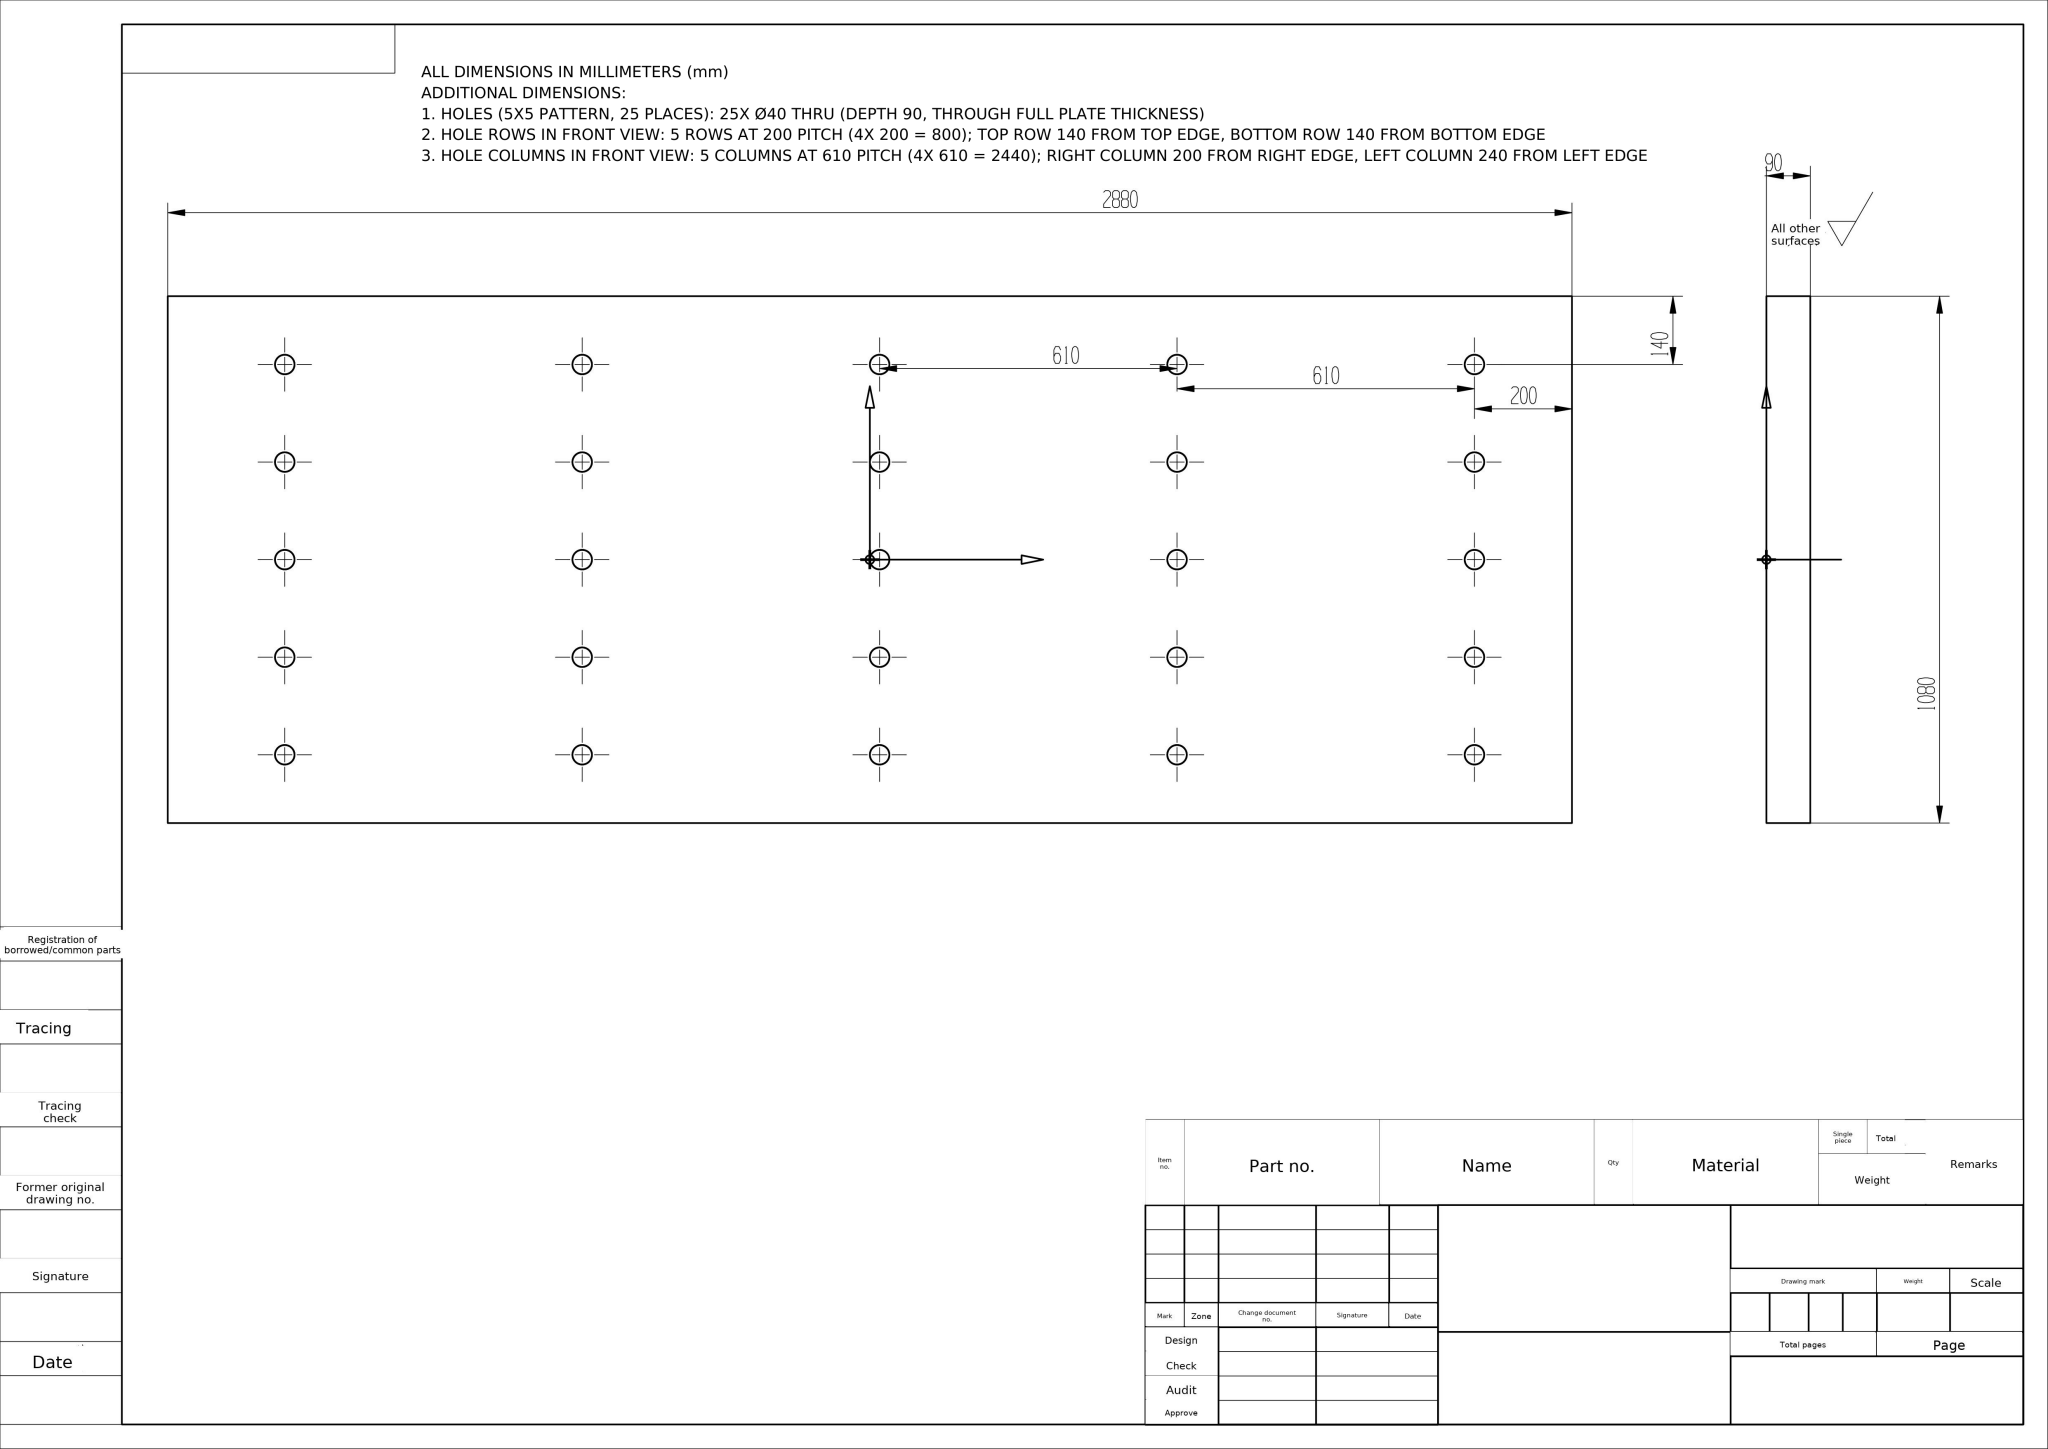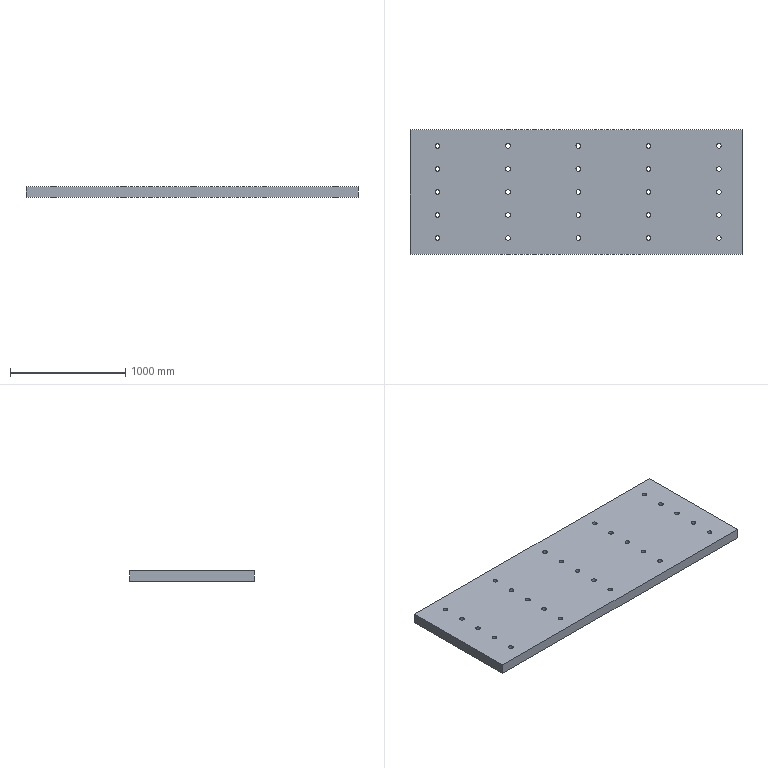Part | NX | mm | 1 solid | 31 faces | box 2880 x 1080 x 90 mm | volume 277108567 mm3 | cylinder 25 | plane 6 | commonest cylinder face diameters 40 x25
STEP:
#1=CARTESIAN_POINT('',(0.,0.,0.));
#2=DIRECTION('',(0.,0.,1.));
#3=DIRECTION('',(1.,0.,0.));
#4=AXIS2_PLACEMENT_3D('',#1,#2,#3);
#5=(LENGTH_UNIT()NAMED_UNIT(*)SI_UNIT(.MILLI.,.METRE.));
#6=UNCERTAINTY_MEASURE_WITH_UNIT(LENGTH_MEASURE(0.00002),#5,'','');
#7=(NAMED_UNIT(*)PLANE_ANGLE_UNIT()SI_UNIT($,.RADIAN.));
#8=PLANE_ANGLE_MEASURE_WITH_UNIT(PLANE_ANGLE_MEASURE(0.01745),#7);
#9=DIMENSIONAL_EXPONENTS(0.,0.,0.,0.,0.,0.,0.);
#10=(CONVERSION_BASED_UNIT('',#8)NAMED_UNIT(#9)PLANE_ANGLE_UNIT());
#11=(NAMED_UNIT(*)SI_UNIT($,.STERADIAN.)SOLID_ANGLE_UNIT());
#12=(GEOMETRIC_REPRESENTATION_CONTEXT(3)GLOBAL_UNCERTAINTY_ASSIGNED_CONTEXT((#6))GLOBAL_UNIT_ASSIGNED_CONTEXT((#5,#10,#11))REPRESENTATION_CONTEXT('',''));
#13=SHAPE_REPRESENTATION('',(#4),#12);
#14=CARTESIAN_POINT('',(-1440.,540.,0.));
#15=VERTEX_POINT('',#14);
#16=CARTESIAN_POINT('',(-1440.,-540.,0.));
#17=VERTEX_POINT('',#16);
#18=CARTESIAN_POINT('',(-1440.,540.,0.));
#19=DIRECTION('',(-0.,-1.,0.));
#20=VECTOR('',#19,1.);
#21=LINE('',#18,#20);
#22=EDGE_CURVE('',#15,#17,#21,.T.);
#23=ORIENTED_EDGE('',*,*,#22,.T.);
#24=CARTESIAN_POINT('',(-1440.,-540.,90.));
#25=VERTEX_POINT('',#24);
#26=CARTESIAN_POINT('',(-1440.,-540.,90.));
#27=DIRECTION('',(0.,0.,-1.));
#28=VECTOR('',#27,1.);
#29=LINE('',#26,#28);
#30=EDGE_CURVE('',#25,#17,#29,.T.);
#31=ORIENTED_EDGE('',*,*,#30,.F.);
#32=CARTESIAN_POINT('',(-1440.,540.,90.));
#33=VERTEX_POINT('',#32);
#34=CARTESIAN_POINT('',(-1440.,540.,90.));
#35=DIRECTION('',(-0.,-1.,0.));
#36=VECTOR('',#35,1.);
#37=LINE('',#34,#36);
#38=EDGE_CURVE('',#33,#25,#37,.T.);
#39=ORIENTED_EDGE('',*,*,#38,.F.);
#40=CARTESIAN_POINT('',(-1440.,540.,90.));
#41=DIRECTION('',(0.,0.,-1.));
#42=VECTOR('',#41,1.);
#43=LINE('',#40,#42);
#44=EDGE_CURVE('',#33,#15,#43,.T.);
#45=ORIENTED_EDGE('',*,*,#44,.T.);
#46=EDGE_LOOP('',(#23,#31,#39,#45));
#47=FACE_OUTER_BOUND('',#46,.T.);
#48=CARTESIAN_POINT('',(-1440.,540.,90.));
#49=DIRECTION('',(1.,-0.,0.));
#50=DIRECTION('',(0.,1.,0.));
#51=AXIS2_PLACEMENT_3D('',#48,#49,#50);
#52=PLANE('',#51);
#53=ADVANCED_FACE('',(#47),#52,.F.);
#54=CARTESIAN_POINT('',(1440.,-540.,0.));
#55=VERTEX_POINT('',#54);
#56=CARTESIAN_POINT('',(-1440.,-540.,0.));
#57=DIRECTION('',(1.,0.,0.));
#58=VECTOR('',#57,1.);
#59=LINE('',#56,#58);
#60=EDGE_CURVE('',#17,#55,#59,.T.);
#61=ORIENTED_EDGE('',*,*,#60,.T.);
#62=CARTESIAN_POINT('',(1440.,-540.,90.));
#63=VERTEX_POINT('',#62);
#64=CARTESIAN_POINT('',(1440.,-540.,90.));
#65=DIRECTION('',(0.,0.,-1.));
#66=VECTOR('',#65,1.);
#67=LINE('',#64,#66);
#68=EDGE_CURVE('',#63,#55,#67,.T.);
#69=ORIENTED_EDGE('',*,*,#68,.F.);
#70=CARTESIAN_POINT('',(-1440.,-540.,90.));
#71=DIRECTION('',(1.,0.,0.));
#72=VECTOR('',#71,1.);
#73=LINE('',#70,#72);
#74=EDGE_CURVE('',#25,#63,#73,.T.);
#75=ORIENTED_EDGE('',*,*,#74,.F.);
#76=ORIENTED_EDGE('',*,*,#30,.T.);
#77=EDGE_LOOP('',(#61,#69,#75,#76));
#78=FACE_OUTER_BOUND('',#77,.T.);
#79=CARTESIAN_POINT('',(-1440.,-540.,90.));
#80=DIRECTION('',(0.,1.,0.));
#81=DIRECTION('',(0.,0.,1.));
#82=AXIS2_PLACEMENT_3D('',#79,#80,#81);
#83=PLANE('',#82);
#84=ADVANCED_FACE('',(#78),#83,.F.);
#85=CARTESIAN_POINT('',(1440.,540.,0.));
#86=VERTEX_POINT('',#85);
#87=CARTESIAN_POINT('',(1440.,-540.,0.));
#88=DIRECTION('',(0.,1.,0.));
#89=VECTOR('',#88,1.);
#90=LINE('',#87,#89);
#91=EDGE_CURVE('',#55,#86,#90,.T.);
#92=ORIENTED_EDGE('',*,*,#91,.T.);
#93=CARTESIAN_POINT('',(1440.,540.,90.));
#94=VERTEX_POINT('',#93);
#95=CARTESIAN_POINT('',(1440.,540.,90.));
#96=DIRECTION('',(0.,0.,-1.));
#97=VECTOR('',#96,1.);
#98=LINE('',#95,#97);
#99=EDGE_CURVE('',#94,#86,#98,.T.);
#100=ORIENTED_EDGE('',*,*,#99,.F.);
#101=CARTESIAN_POINT('',(1440.,-540.,90.));
#102=DIRECTION('',(0.,1.,0.));
#103=VECTOR('',#102,1.);
#104=LINE('',#101,#103);
#105=EDGE_CURVE('',#63,#94,#104,.T.);
#106=ORIENTED_EDGE('',*,*,#105,.F.);
#107=ORIENTED_EDGE('',*,*,#68,.T.);
#108=EDGE_LOOP('',(#92,#100,#106,#107));
#109=FACE_OUTER_BOUND('',#108,.T.);
#110=CARTESIAN_POINT('',(1440.,-540.,90.));
#111=DIRECTION('',(-1.,0.,0.));
#112=DIRECTION('',(0.,0.,1.));
#113=AXIS2_PLACEMENT_3D('',#110,#111,#112);
#114=PLANE('',#113);
#115=ADVANCED_FACE('',(#109),#114,.F.);
#116=CARTESIAN_POINT('',(1260.,200.,90.));
#117=VERTEX_POINT('',#116);
#118=CARTESIAN_POINT('',(1240.,200.,90.));
#119=DIRECTION('',(0.,0.,1.));
#120=DIRECTION('',(1.,0.,0.));
#121=AXIS2_PLACEMENT_3D('',#118,#119,#120);
#122=CIRCLE('',#121,20.);
#123=EDGE_CURVE('',#117,#117,#122,.T.);
#124=ORIENTED_EDGE('',*,*,#123,.T.);
#125=EDGE_LOOP('',(#124));
#126=FACE_BOUND('',#125,.T.);
#127=CARTESIAN_POINT('',(1260.,200.,0.));
#128=VERTEX_POINT('',#127);
#129=CARTESIAN_POINT('',(1240.,200.,0.));
#130=DIRECTION('',(0.,0.,1.));
#131=DIRECTION('',(1.,0.,0.));
#132=AXIS2_PLACEMENT_3D('',#129,#130,#131);
#133=CIRCLE('',#132,20.);
#134=EDGE_CURVE('',#128,#128,#133,.T.);
#135=ORIENTED_EDGE('',*,*,#134,.F.);
#136=EDGE_LOOP('',(#135));
#137=FACE_BOUND('',#136,.T.);
#138=CARTESIAN_POINT('',(1240.,200.,90.));
#139=DIRECTION('',(0.,0.,-1.));
#140=DIRECTION('',(-1.,0.,0.));
#141=AXIS2_PLACEMENT_3D('',#138,#139,#140);
#142=CYLINDRICAL_SURFACE('',#141,20.);
#143=ADVANCED_FACE('',(#126,#137),#142,.F.);
#144=CARTESIAN_POINT('',(1260.,-0.,90.));
#145=VERTEX_POINT('',#144);
#146=CARTESIAN_POINT('',(1240.,-0.,90.));
#147=DIRECTION('',(0.,0.,1.));
#148=DIRECTION('',(1.,0.,0.));
#149=AXIS2_PLACEMENT_3D('',#146,#147,#148);
#150=CIRCLE('',#149,20.);
#151=EDGE_CURVE('',#145,#145,#150,.T.);
#152=ORIENTED_EDGE('',*,*,#151,.T.);
#153=EDGE_LOOP('',(#152));
#154=FACE_BOUND('',#153,.T.);
#155=CARTESIAN_POINT('',(1260.,-0.,0.));
#156=VERTEX_POINT('',#155);
#157=CARTESIAN_POINT('',(1240.,-0.,0.));
#158=DIRECTION('',(0.,0.,1.));
#159=DIRECTION('',(1.,0.,0.));
#160=AXIS2_PLACEMENT_3D('',#157,#158,#159);
#161=CIRCLE('',#160,20.);
#162=EDGE_CURVE('',#156,#156,#161,.T.);
#163=ORIENTED_EDGE('',*,*,#162,.F.);
#164=EDGE_LOOP('',(#163));
#165=FACE_BOUND('',#164,.T.);
#166=CARTESIAN_POINT('',(1240.,-0.,90.));
#167=DIRECTION('',(0.,0.,-1.));
#168=DIRECTION('',(-1.,0.,0.));
#169=AXIS2_PLACEMENT_3D('',#166,#167,#168);
#170=CYLINDRICAL_SURFACE('',#169,20.);
#171=ADVANCED_FACE('',(#154,#165),#170,.F.);
#172=CARTESIAN_POINT('',(1260.,-200.,90.));
#173=VERTEX_POINT('',#172);
#174=CARTESIAN_POINT('',(1240.,-200.,90.));
#175=DIRECTION('',(0.,0.,1.));
#176=DIRECTION('',(1.,0.,0.));
#177=AXIS2_PLACEMENT_3D('',#174,#175,#176);
#178=CIRCLE('',#177,20.);
#179=EDGE_CURVE('',#173,#173,#178,.T.);
#180=ORIENTED_EDGE('',*,*,#179,.T.);
#181=EDGE_LOOP('',(#180));
#182=FACE_BOUND('',#181,.T.);
#183=CARTESIAN_POINT('',(1260.,-200.,0.));
#184=VERTEX_POINT('',#183);
#185=CARTESIAN_POINT('',(1240.,-200.,0.));
#186=DIRECTION('',(0.,0.,1.));
#187=DIRECTION('',(1.,0.,0.));
#188=AXIS2_PLACEMENT_3D('',#185,#186,#187);
#189=CIRCLE('',#188,20.);
#190=EDGE_CURVE('',#184,#184,#189,.T.);
#191=ORIENTED_EDGE('',*,*,#190,.F.);
#192=EDGE_LOOP('',(#191));
#193=FACE_BOUND('',#192,.T.);
#194=CARTESIAN_POINT('',(1240.,-200.,90.));
#195=DIRECTION('',(0.,0.,-1.));
#196=DIRECTION('',(-1.,0.,0.));
#197=AXIS2_PLACEMENT_3D('',#194,#195,#196);
#198=CYLINDRICAL_SURFACE('',#197,20.);
#199=ADVANCED_FACE('',(#182,#193),#198,.F.);
#200=CARTESIAN_POINT('',(1260.,-400.,90.));
#201=VERTEX_POINT('',#200);
#202=CARTESIAN_POINT('',(1240.,-400.,90.));
#203=DIRECTION('',(0.,0.,1.));
#204=DIRECTION('',(1.,0.,0.));
#205=AXIS2_PLACEMENT_3D('',#202,#203,#204);
#206=CIRCLE('',#205,20.);
#207=EDGE_CURVE('',#201,#201,#206,.T.);
#208=ORIENTED_EDGE('',*,*,#207,.T.);
#209=EDGE_LOOP('',(#208));
#210=FACE_BOUND('',#209,.T.);
#211=CARTESIAN_POINT('',(1260.,-400.,0.));
#212=VERTEX_POINT('',#211);
#213=CARTESIAN_POINT('',(1240.,-400.,0.));
#214=DIRECTION('',(0.,0.,1.));
#215=DIRECTION('',(1.,0.,0.));
#216=AXIS2_PLACEMENT_3D('',#213,#214,#215);
#217=CIRCLE('',#216,20.);
#218=EDGE_CURVE('',#212,#212,#217,.T.);
#219=ORIENTED_EDGE('',*,*,#218,.F.);
#220=EDGE_LOOP('',(#219));
#221=FACE_BOUND('',#220,.T.);
#222=CARTESIAN_POINT('',(1240.,-400.,90.));
#223=DIRECTION('',(0.,0.,-1.));
#224=DIRECTION('',(-1.,0.,0.));
#225=AXIS2_PLACEMENT_3D('',#222,#223,#224);
#226=CYLINDRICAL_SURFACE('',#225,20.);
#227=ADVANCED_FACE('',(#210,#221),#226,.F.);
#228=CARTESIAN_POINT('',(650.,400.,90.));
#229=VERTEX_POINT('',#228);
#230=CARTESIAN_POINT('',(630.,400.,90.));
#231=DIRECTION('',(0.,0.,1.));
#232=DIRECTION('',(1.,0.,0.));
#233=AXIS2_PLACEMENT_3D('',#230,#231,#232);
#234=CIRCLE('',#233,20.);
#235=EDGE_CURVE('',#229,#229,#234,.T.);
#236=ORIENTED_EDGE('',*,*,#235,.T.);
#237=EDGE_LOOP('',(#236));
#238=FACE_BOUND('',#237,.T.);
#239=CARTESIAN_POINT('',(650.,400.,0.));
#240=VERTEX_POINT('',#239);
#241=CARTESIAN_POINT('',(630.,400.,0.));
#242=DIRECTION('',(0.,0.,1.));
#243=DIRECTION('',(1.,0.,0.));
#244=AXIS2_PLACEMENT_3D('',#241,#242,#243);
#245=CIRCLE('',#244,20.);
#246=EDGE_CURVE('',#240,#240,#245,.T.);
#247=ORIENTED_EDGE('',*,*,#246,.F.);
#248=EDGE_LOOP('',(#247));
#249=FACE_BOUND('',#248,.T.);
#250=CARTESIAN_POINT('',(630.,400.,90.));
#251=DIRECTION('',(0.,0.,-1.));
#252=DIRECTION('',(-1.,0.,0.));
#253=AXIS2_PLACEMENT_3D('',#250,#251,#252);
#254=CYLINDRICAL_SURFACE('',#253,20.);
#255=ADVANCED_FACE('',(#238,#249),#254,.F.);
#256=CARTESIAN_POINT('',(650.,200.,90.));
#257=VERTEX_POINT('',#256);
#258=CARTESIAN_POINT('',(630.,200.,90.));
#259=DIRECTION('',(0.,0.,1.));
#260=DIRECTION('',(1.,0.,0.));
#261=AXIS2_PLACEMENT_3D('',#258,#259,#260);
#262=CIRCLE('',#261,20.);
#263=EDGE_CURVE('',#257,#257,#262,.T.);
#264=ORIENTED_EDGE('',*,*,#263,.T.);
#265=EDGE_LOOP('',(#264));
#266=FACE_BOUND('',#265,.T.);
#267=CARTESIAN_POINT('',(650.,200.,0.));
#268=VERTEX_POINT('',#267);
#269=CARTESIAN_POINT('',(630.,200.,0.));
#270=DIRECTION('',(0.,0.,1.));
#271=DIRECTION('',(1.,0.,0.));
#272=AXIS2_PLACEMENT_3D('',#269,#270,#271);
#273=CIRCLE('',#272,20.);
#274=EDGE_CURVE('',#268,#268,#273,.T.);
#275=ORIENTED_EDGE('',*,*,#274,.F.);
#276=EDGE_LOOP('',(#275));
#277=FACE_BOUND('',#276,.T.);
#278=CARTESIAN_POINT('',(630.,200.,90.));
#279=DIRECTION('',(0.,0.,-1.));
#280=DIRECTION('',(-1.,0.,0.));
#281=AXIS2_PLACEMENT_3D('',#278,#279,#280);
#282=CYLINDRICAL_SURFACE('',#281,20.);
#283=ADVANCED_FACE('',(#266,#277),#282,.F.);
#284=CARTESIAN_POINT('',(650.,-0.,90.));
#285=VERTEX_POINT('',#284);
#286=CARTESIAN_POINT('',(630.,-0.,90.));
#287=DIRECTION('',(0.,0.,1.));
#288=DIRECTION('',(1.,0.,0.));
#289=AXIS2_PLACEMENT_3D('',#286,#287,#288);
#290=CIRCLE('',#289,20.);
#291=EDGE_CURVE('',#285,#285,#290,.T.);
#292=ORIENTED_EDGE('',*,*,#291,.T.);
#293=EDGE_LOOP('',(#292));
#294=FACE_BOUND('',#293,.T.);
#295=CARTESIAN_POINT('',(650.,-0.,0.));
#296=VERTEX_POINT('',#295);
#297=CARTESIAN_POINT('',(630.,-0.,0.));
#298=DIRECTION('',(0.,0.,1.));
#299=DIRECTION('',(1.,0.,0.));
#300=AXIS2_PLACEMENT_3D('',#297,#298,#299);
#301=CIRCLE('',#300,20.);
#302=EDGE_CURVE('',#296,#296,#301,.T.);
#303=ORIENTED_EDGE('',*,*,#302,.F.);
#304=EDGE_LOOP('',(#303));
#305=FACE_BOUND('',#304,.T.);
#306=CARTESIAN_POINT('',(630.,-0.,90.));
#307=DIRECTION('',(0.,0.,-1.));
#308=DIRECTION('',(-1.,0.,0.));
#309=AXIS2_PLACEMENT_3D('',#306,#307,#308);
#310=CYLINDRICAL_SURFACE('',#309,20.);
#311=ADVANCED_FACE('',(#294,#305),#310,.F.);
#312=CARTESIAN_POINT('',(650.,-200.,90.));
#313=VERTEX_POINT('',#312);
#314=CARTESIAN_POINT('',(630.,-200.,90.));
#315=DIRECTION('',(0.,0.,1.));
#316=DIRECTION('',(1.,0.,0.));
#317=AXIS2_PLACEMENT_3D('',#314,#315,#316);
#318=CIRCLE('',#317,20.);
#319=EDGE_CURVE('',#313,#313,#318,.T.);
#320=ORIENTED_EDGE('',*,*,#319,.T.);
#321=EDGE_LOOP('',(#320));
#322=FACE_BOUND('',#321,.T.);
#323=CARTESIAN_POINT('',(650.,-200.,0.));
#324=VERTEX_POINT('',#323);
#325=CARTESIAN_POINT('',(630.,-200.,0.));
#326=DIRECTION('',(0.,0.,1.));
#327=DIRECTION('',(1.,0.,0.));
#328=AXIS2_PLACEMENT_3D('',#325,#326,#327);
#329=CIRCLE('',#328,20.);
#330=EDGE_CURVE('',#324,#324,#329,.T.);
#331=ORIENTED_EDGE('',*,*,#330,.F.);
#332=EDGE_LOOP('',(#331));
#333=FACE_BOUND('',#332,.T.);
#334=CARTESIAN_POINT('',(630.,-200.,90.));
#335=DIRECTION('',(0.,0.,-1.));
#336=DIRECTION('',(-1.,0.,0.));
#337=AXIS2_PLACEMENT_3D('',#334,#335,#336);
#338=CYLINDRICAL_SURFACE('',#337,20.);
#339=ADVANCED_FACE('',(#322,#333),#338,.F.);
#340=CARTESIAN_POINT('',(650.,-400.,90.));
#341=VERTEX_POINT('',#340);
#342=CARTESIAN_POINT('',(630.,-400.,90.));
#343=DIRECTION('',(0.,0.,1.));
#344=DIRECTION('',(1.,0.,0.));
#345=AXIS2_PLACEMENT_3D('',#342,#343,#344);
#346=CIRCLE('',#345,20.);
#347=EDGE_CURVE('',#341,#341,#346,.T.);
#348=ORIENTED_EDGE('',*,*,#347,.T.);
#349=EDGE_LOOP('',(#348));
#350=FACE_BOUND('',#349,.T.);
#351=CARTESIAN_POINT('',(650.,-400.,0.));
#352=VERTEX_POINT('',#351);
#353=CARTESIAN_POINT('',(630.,-400.,0.));
#354=DIRECTION('',(0.,0.,1.));
#355=DIRECTION('',(1.,0.,0.));
#356=AXIS2_PLACEMENT_3D('',#353,#354,#355);
#357=CIRCLE('',#356,20.);
#358=EDGE_CURVE('',#352,#352,#357,.T.);
#359=ORIENTED_EDGE('',*,*,#358,.F.);
#360=EDGE_LOOP('',(#359));
#361=FACE_BOUND('',#360,.T.);
#362=CARTESIAN_POINT('',(630.,-400.,90.));
#363=DIRECTION('',(0.,0.,-1.));
#364=DIRECTION('',(-1.,0.,0.));
#365=AXIS2_PLACEMENT_3D('',#362,#363,#364);
#366=CYLINDRICAL_SURFACE('',#365,20.);
#367=ADVANCED_FACE('',(#350,#361),#366,.F.);
#368=CARTESIAN_POINT('',(40.,400.,90.));
#369=VERTEX_POINT('',#368);
#370=CARTESIAN_POINT('',(20.,400.,90.));
#371=DIRECTION('',(0.,0.,1.));
#372=DIRECTION('',(1.,0.,0.));
#373=AXIS2_PLACEMENT_3D('',#370,#371,#372);
#374=CIRCLE('',#373,20.);
#375=EDGE_CURVE('',#369,#369,#374,.T.);
#376=ORIENTED_EDGE('',*,*,#375,.T.);
#377=EDGE_LOOP('',(#376));
#378=FACE_BOUND('',#377,.T.);
#379=CARTESIAN_POINT('',(40.,400.,0.));
#380=VERTEX_POINT('',#379);
#381=CARTESIAN_POINT('',(20.,400.,0.));
#382=DIRECTION('',(0.,0.,1.));
#383=DIRECTION('',(1.,0.,0.));
#384=AXIS2_PLACEMENT_3D('',#381,#382,#383);
#385=CIRCLE('',#384,20.);
#386=EDGE_CURVE('',#380,#380,#385,.T.);
#387=ORIENTED_EDGE('',*,*,#386,.F.);
#388=EDGE_LOOP('',(#387));
#389=FACE_BOUND('',#388,.T.);
#390=CARTESIAN_POINT('',(20.,400.,90.));
#391=DIRECTION('',(0.,0.,-1.));
#392=DIRECTION('',(-1.,0.,0.));
#393=AXIS2_PLACEMENT_3D('',#390,#391,#392);
#394=CYLINDRICAL_SURFACE('',#393,20.);
#395=ADVANCED_FACE('',(#378,#389),#394,.F.);
#396=CARTESIAN_POINT('',(40.,200.,90.));
#397=VERTEX_POINT('',#396);
#398=CARTESIAN_POINT('',(20.,200.,90.));
#399=DIRECTION('',(0.,0.,1.));
#400=DIRECTION('',(1.,0.,0.));
#401=AXIS2_PLACEMENT_3D('',#398,#399,#400);
#402=CIRCLE('',#401,20.);
#403=EDGE_CURVE('',#397,#397,#402,.T.);
#404=ORIENTED_EDGE('',*,*,#403,.T.);
#405=EDGE_LOOP('',(#404));
#406=FACE_BOUND('',#405,.T.);
#407=CARTESIAN_POINT('',(40.,200.,0.));
#408=VERTEX_POINT('',#407);
#409=CARTESIAN_POINT('',(20.,200.,0.));
#410=DIRECTION('',(0.,0.,1.));
#411=DIRECTION('',(1.,0.,0.));
#412=AXIS2_PLACEMENT_3D('',#409,#410,#411);
#413=CIRCLE('',#412,20.);
#414=EDGE_CURVE('',#408,#408,#413,.T.);
#415=ORIENTED_EDGE('',*,*,#414,.F.);
#416=EDGE_LOOP('',(#415));
#417=FACE_BOUND('',#416,.T.);
#418=CARTESIAN_POINT('',(20.,200.,90.));
#419=DIRECTION('',(0.,0.,-1.));
#420=DIRECTION('',(-1.,0.,0.));
#421=AXIS2_PLACEMENT_3D('',#418,#419,#420);
#422=CYLINDRICAL_SURFACE('',#421,20.);
#423=ADVANCED_FACE('',(#406,#417),#422,.F.);
#424=CARTESIAN_POINT('',(40.,-0.,90.));
#425=VERTEX_POINT('',#424);
#426=CARTESIAN_POINT('',(20.,-0.,90.));
#427=DIRECTION('',(0.,0.,1.));
#428=DIRECTION('',(1.,0.,0.));
#429=AXIS2_PLACEMENT_3D('',#426,#427,#428);
#430=CIRCLE('',#429,20.);
#431=EDGE_CURVE('',#425,#425,#430,.T.);
#432=ORIENTED_EDGE('',*,*,#431,.T.);
#433=EDGE_LOOP('',(#432));
#434=FACE_BOUND('',#433,.T.);
#435=CARTESIAN_POINT('',(40.,-0.,0.));
#436=VERTEX_POINT('',#435);
#437=CARTESIAN_POINT('',(20.,-0.,0.));
#438=DIRECTION('',(0.,0.,1.));
#439=DIRECTION('',(1.,0.,0.));
#440=AXIS2_PLACEMENT_3D('',#437,#438,#439);
#441=CIRCLE('',#440,20.);
#442=EDGE_CURVE('',#436,#436,#441,.T.);
#443=ORIENTED_EDGE('',*,*,#442,.F.);
#444=EDGE_LOOP('',(#443));
#445=FACE_BOUND('',#444,.T.);
#446=CARTESIAN_POINT('',(20.,-0.,90.));
#447=DIRECTION('',(0.,0.,-1.));
#448=DIRECTION('',(-1.,0.,0.));
#449=AXIS2_PLACEMENT_3D('',#446,#447,#448);
#450=CYLINDRICAL_SURFACE('',#449,20.);
#451=ADVANCED_FACE('',(#434,#445),#450,.F.);
#452=CARTESIAN_POINT('',(40.,-200.,90.));
#453=VERTEX_POINT('',#452);
#454=CARTESIAN_POINT('',(20.,-200.,90.));
#455=DIRECTION('',(0.,0.,1.));
#456=DIRECTION('',(1.,0.,0.));
#457=AXIS2_PLACEMENT_3D('',#454,#455,#456);
#458=CIRCLE('',#457,20.);
#459=EDGE_CURVE('',#453,#453,#458,.T.);
#460=ORIENTED_EDGE('',*,*,#459,.T.);
#461=EDGE_LOOP('',(#460));
#462=FACE_BOUND('',#461,.T.);
#463=CARTESIAN_POINT('',(40.,-200.,0.));
#464=VERTEX_POINT('',#463);
#465=CARTESIAN_POINT('',(20.,-200.,0.));
#466=DIRECTION('',(0.,0.,1.));
#467=DIRECTION('',(1.,0.,0.));
#468=AXIS2_PLACEMENT_3D('',#465,#466,#467);
#469=CIRCLE('',#468,20.);
#470=EDGE_CURVE('',#464,#464,#469,.T.);
#471=ORIENTED_EDGE('',*,*,#470,.F.);
#472=EDGE_LOOP('',(#471));
#473=FACE_BOUND('',#472,.T.);
#474=CARTESIAN_POINT('',(20.,-200.,90.));
#475=DIRECTION('',(0.,0.,-1.));
#476=DIRECTION('',(-1.,0.,0.));
#477=AXIS2_PLACEMENT_3D('',#474,#475,#476);
#478=CYLINDRICAL_SURFACE('',#477,20.);
#479=ADVANCED_FACE('',(#462,#473),#478,.F.);
#480=CARTESIAN_POINT('',(40.,-400.,90.));
#481=VERTEX_POINT('',#480);
#482=CARTESIAN_POINT('',(20.,-400.,90.));
#483=DIRECTION('',(0.,0.,1.));
#484=DIRECTION('',(1.,0.,0.));
#485=AXIS2_PLACEMENT_3D('',#482,#483,#484);
#486=CIRCLE('',#485,20.);
#487=EDGE_CURVE('',#481,#481,#486,.T.);
#488=ORIENTED_EDGE('',*,*,#487,.T.);
#489=EDGE_LOOP('',(#488));
#490=FACE_BOUND('',#489,.T.);
#491=CARTESIAN_POINT('',(40.,-400.,0.));
#492=VERTEX_POINT('',#491);
#493=CARTESIAN_POINT('',(20.,-400.,0.));
#494=DIRECTION('',(0.,0.,1.));
#495=DIRECTION('',(1.,0.,0.));
#496=AXIS2_PLACEMENT_3D('',#493,#494,#495);
#497=CIRCLE('',#496,20.);
#498=EDGE_CURVE('',#492,#492,#497,.T.);
#499=ORIENTED_EDGE('',*,*,#498,.F.);
#500=EDGE_LOOP('',(#499));
#501=FACE_BOUND('',#500,.T.);
#502=CARTESIAN_POINT('',(20.,-400.,90.));
#503=DIRECTION('',(0.,0.,-1.));
#504=DIRECTION('',(-1.,0.,0.));
#505=AXIS2_PLACEMENT_3D('',#502,#503,#504);
#506=CYLINDRICAL_SURFACE('',#505,20.);
#507=ADVANCED_FACE('',(#490,#501),#506,.F.);
#508=CARTESIAN_POINT('',(-570.,400.,90.));
#509=VERTEX_POINT('',#508);
#510=CARTESIAN_POINT('',(-590.,400.,90.));
#511=DIRECTION('',(0.,0.,1.));
#512=DIRECTION('',(1.,0.,0.));
#513=AXIS2_PLACEMENT_3D('',#510,#511,#512);
#514=CIRCLE('',#513,20.);
#515=EDGE_CURVE('',#509,#509,#514,.T.);
#516=ORIENTED_EDGE('',*,*,#515,.T.);
#517=EDGE_LOOP('',(#516));
#518=FACE_BOUND('',#517,.T.);
#519=CARTESIAN_POINT('',(-570.,400.,0.));
#520=VERTEX_POINT('',#519);
#521=CARTESIAN_POINT('',(-590.,400.,0.));
#522=DIRECTION('',(0.,0.,1.));
#523=DIRECTION('',(1.,0.,0.));
#524=AXIS2_PLACEMENT_3D('',#521,#522,#523);
#525=CIRCLE('',#524,20.);
#526=EDGE_CURVE('',#520,#520,#525,.T.);
#527=ORIENTED_EDGE('',*,*,#526,.F.);
#528=EDGE_LOOP('',(#527));
#529=FACE_BOUND('',#528,.T.);
#530=CARTESIAN_POINT('',(-590.,400.,90.));
#531=DIRECTION('',(0.,0.,-1.));
#532=DIRECTION('',(-1.,0.,0.));
#533=AXIS2_PLACEMENT_3D('',#530,#531,#532);
#534=CYLINDRICAL_SURFACE('',#533,20.);
#535=ADVANCED_FACE('',(#518,#529),#534,.F.);
#536=CARTESIAN_POINT('',(-570.,200.,90.));
#537=VERTEX_POINT('',#536);
#538=CARTESIAN_POINT('',(-590.,200.,90.));
#539=DIRECTION('',(0.,0.,1.));
#540=DIRECTION('',(1.,0.,0.));
#541=AXIS2_PLACEMENT_3D('',#538,#539,#540);
#542=CIRCLE('',#541,20.);
#543=EDGE_CURVE('',#537,#537,#542,.T.);
#544=ORIENTED_EDGE('',*,*,#543,.T.);
#545=EDGE_LOOP('',(#544));
#546=FACE_BOUND('',#545,.T.);
#547=CARTESIAN_POINT('',(-570.,200.,0.));
#548=VERTEX_POINT('',#547);
#549=CARTESIAN_POINT('',(-590.,200.,0.));
#550=DIRECTION('',(0.,0.,1.));
#551=DIRECTION('',(1.,0.,0.));
#552=AXIS2_PLACEMENT_3D('',#549,#550,#551);
#553=CIRCLE('',#552,20.);
#554=EDGE_CURVE('',#548,#548,#553,.T.);
#555=ORIENTED_EDGE('',*,*,#554,.F.);
#556=EDGE_LOOP('',(#555));
#557=FACE_BOUND('',#556,.T.);
#558=CARTESIAN_POINT('',(-590.,200.,90.));
#559=DIRECTION('',(0.,0.,-1.));
#560=DIRECTION('',(-1.,0.,0.));
#561=AXIS2_PLACEMENT_3D('',#558,#559,#560);
#562=CYLINDRICAL_SURFACE('',#561,20.);
#563=ADVANCED_FACE('',(#546,#557),#562,.F.);
#564=CARTESIAN_POINT('',(-570.,-0.,90.));
#565=VERTEX_POINT('',#564);
#566=CARTESIAN_POINT('',(-590.,-0.,90.));
#567=DIRECTION('',(0.,0.,1.));
#568=DIRECTION('',(1.,0.,0.));
#569=AXIS2_PLACEMENT_3D('',#566,#567,#568);
#570=CIRCLE('',#569,20.);
#571=EDGE_CURVE('',#565,#565,#570,.T.);
#572=ORIENTED_EDGE('',*,*,#571,.T.);
#573=EDGE_LOOP('',(#572));
#574=FACE_BOUND('',#573,.T.);
#575=CARTESIAN_POINT('',(-570.,-0.,0.));
#576=VERTEX_POINT('',#575);
#577=CARTESIAN_POINT('',(-590.,-0.,0.));
#578=DIRECTION('',(0.,0.,1.));
#579=DIRECTION('',(1.,0.,0.));
#580=AXIS2_PLACEMENT_3D('',#577,#578,#579);
#581=CIRCLE('',#580,20.);
#582=EDGE_CURVE('',#576,#576,#581,.T.);
#583=ORIENTED_EDGE('',*,*,#582,.F.);
#584=EDGE_LOOP('',(#583));
#585=FACE_BOUND('',#584,.T.);
#586=CARTESIAN_POINT('',(-590.,-0.,90.));
#587=DIRECTION('',(0.,0.,-1.));
#588=DIRECTION('',(-1.,0.,0.));
#589=AXIS2_PLACEMENT_3D('',#586,#587,#588);
#590=CYLINDRICAL_SURFACE('',#589,20.);
#591=ADVANCED_FACE('',(#574,#585),#590,.F.);
#592=CARTESIAN_POINT('',(-570.,-200.,90.));
#593=VERTEX_POINT('',#592);
#594=CARTESIAN_POINT('',(-590.,-200.,90.));
#595=DIRECTION('',(0.,0.,1.));
#596=DIRECTION('',(1.,0.,0.));
#597=AXIS2_PLACEMENT_3D('',#594,#595,#596);
#598=CIRCLE('',#597,20.);
#599=EDGE_CURVE('',#593,#593,#598,.T.);
#600=ORIENTED_EDGE('',*,*,#599,.T.);
#601=EDGE_LOOP('',(#600));
#602=FACE_BOUND('',#601,.T.);
#603=CARTESIAN_POINT('',(-570.,-200.,0.));
#604=VERTEX_POINT('',#603);
#605=CARTESIAN_POINT('',(-590.,-200.,0.));
#606=DIRECTION('',(0.,0.,1.));
#607=DIRECTION('',(1.,0.,0.));
#608=AXIS2_PLACEMENT_3D('',#605,#606,#607);
#609=CIRCLE('',#608,20.);
#610=EDGE_CURVE('',#604,#604,#609,.T.);
#611=ORIENTED_EDGE('',*,*,#610,.F.);
#612=EDGE_LOOP('',(#611));
#613=FACE_BOUND('',#612,.T.);
#614=CARTESIAN_POINT('',(-590.,-200.,90.));
#615=DIRECTION('',(0.,0.,-1.));
#616=DIRECTION('',(-1.,0.,0.));
#617=AXIS2_PLACEMENT_3D('',#614,#615,#616);
#618=CYLINDRICAL_SURFACE('',#617,20.);
#619=ADVANCED_FACE('',(#602,#613),#618,.F.);
#620=CARTESIAN_POINT('',(-570.,-400.,90.));
#621=VERTEX_POINT('',#620);
#622=CARTESIAN_POINT('',(-590.,-400.,90.));
#623=DIRECTION('',(0.,0.,1.));
#624=DIRECTION('',(1.,0.,0.));
#625=AXIS2_PLACEMENT_3D('',#622,#623,#624);
#626=CIRCLE('',#625,20.);
#627=EDGE_CURVE('',#621,#621,#626,.T.);
#628=ORIENTED_EDGE('',*,*,#627,.T.);
#629=EDGE_LOOP('',(#628));
#630=FACE_BOUND('',#629,.T.);
#631=CARTESIAN_POINT('',(-570.,-400.,0.));
#632=VERTEX_POINT('',#631);
#633=CARTESIAN_POINT('',(-590.,-400.,0.));
#634=DIRECTION('',(0.,0.,1.));
#635=DIRECTION('',(1.,0.,0.));
#636=AXIS2_PLACEMENT_3D('',#633,#634,#635);
#637=CIRCLE('',#636,20.);
#638=EDGE_CURVE('',#632,#632,#637,.T.);
#639=ORIENTED_EDGE('',*,*,#638,.F.);
#640=EDGE_LOOP('',(#639));
#641=FACE_BOUND('',#640,.T.);
#642=CARTESIAN_POINT('',(-590.,-400.,90.));
#643=DIRECTION('',(0.,0.,-1.));
#644=DIRECTION('',(-1.,0.,0.));
#645=AXIS2_PLACEMENT_3D('',#642,#643,#644);
#646=CYLINDRICAL_SURFACE('',#645,20.);
#647=ADVANCED_FACE('',(#630,#641),#646,.F.);
#648=CARTESIAN_POINT('',(-1180.,400.,90.));
#649=VERTEX_POINT('',#648);
#650=CARTESIAN_POINT('',(-1200.,400.,90.));
#651=DIRECTION('',(0.,0.,1.));
#652=DIRECTION('',(1.,0.,0.));
#653=AXIS2_PLACEMENT_3D('',#650,#651,#652);
#654=CIRCLE('',#653,20.);
#655=EDGE_CURVE('',#649,#649,#654,.T.);
#656=ORIENTED_EDGE('',*,*,#655,.T.);
#657=EDGE_LOOP('',(#656));
#658=FACE_BOUND('',#657,.T.);
#659=CARTESIAN_POINT('',(-1180.,400.,0.));
#660=VERTEX_POINT('',#659);
#661=CARTESIAN_POINT('',(-1200.,400.,0.));
#662=DIRECTION('',(0.,0.,1.));
#663=DIRECTION('',(1.,0.,0.));
#664=AXIS2_PLACEMENT_3D('',#661,#662,#663);
#665=CIRCLE('',#664,20.);
#666=EDGE_CURVE('',#660,#660,#665,.T.);
#667=ORIENTED_EDGE('',*,*,#666,.F.);
#668=EDGE_LOOP('',(#667));
#669=FACE_BOUND('',#668,.T.);
#670=CARTESIAN_POINT('',(-1200.,400.,90.));
#671=DIRECTION('',(0.,0.,-1.));
#672=DIRECTION('',(-1.,0.,0.));
#673=AXIS2_PLACEMENT_3D('',#670,#671,#672);
#674=CYLINDRICAL_SURFACE('',#673,20.);
#675=ADVANCED_FACE('',(#658,#669),#674,.F.);
#676=CARTESIAN_POINT('',(-1180.,200.,90.));
#677=VERTEX_POINT('',#676);
#678=CARTESIAN_POINT('',(-1200.,200.,90.));
#679=DIRECTION('',(0.,0.,1.));
#680=DIRECTION('',(1.,0.,0.));
#681=AXIS2_PLACEMENT_3D('',#678,#679,#680);
#682=CIRCLE('',#681,20.);
#683=EDGE_CURVE('',#677,#677,#682,.T.);
#684=ORIENTED_EDGE('',*,*,#683,.T.);
#685=EDGE_LOOP('',(#684));
#686=FACE_BOUND('',#685,.T.);
#687=CARTESIAN_POINT('',(-1180.,200.,0.));
#688=VERTEX_POINT('',#687);
#689=CARTESIAN_POINT('',(-1200.,200.,0.));
#690=DIRECTION('',(0.,0.,1.));
#691=DIRECTION('',(1.,0.,0.));
#692=AXIS2_PLACEMENT_3D('',#689,#690,#691);
#693=CIRCLE('',#692,20.);
#694=EDGE_CURVE('',#688,#688,#693,.T.);
#695=ORIENTED_EDGE('',*,*,#694,.F.);
#696=EDGE_LOOP('',(#695));
#697=FACE_BOUND('',#696,.T.);
#698=CARTESIAN_POINT('',(-1200.,200.,90.));
#699=DIRECTION('',(0.,0.,-1.));
#700=DIRECTION('',(-1.,0.,0.));
#701=AXIS2_PLACEMENT_3D('',#698,#699,#700);
#702=CYLINDRICAL_SURFACE('',#701,20.);
#703=ADVANCED_FACE('',(#686,#697),#702,.F.);
#704=CARTESIAN_POINT('',(-1180.,-0.,90.));
#705=VERTEX_POINT('',#704);
#706=CARTESIAN_POINT('',(-1200.,-0.,90.));
#707=DIRECTION('',(0.,0.,1.));
#708=DIRECTION('',(1.,0.,0.));
#709=AXIS2_PLACEMENT_3D('',#706,#707,#708);
#710=CIRCLE('',#709,20.);
#711=EDGE_CURVE('',#705,#705,#710,.T.);
#712=ORIENTED_EDGE('',*,*,#711,.T.);
#713=EDGE_LOOP('',(#712));
#714=FACE_BOUND('',#713,.T.);
#715=CARTESIAN_POINT('',(-1180.,-0.,0.));
#716=VERTEX_POINT('',#715);
#717=CARTESIAN_POINT('',(-1200.,-0.,0.));
#718=DIRECTION('',(0.,0.,1.));
#719=DIRECTION('',(1.,0.,0.));
#720=AXIS2_PLACEMENT_3D('',#717,#718,#719);
#721=CIRCLE('',#720,20.);
#722=EDGE_CURVE('',#716,#716,#721,.T.);
#723=ORIENTED_EDGE('',*,*,#722,.F.);
#724=EDGE_LOOP('',(#723));
#725=FACE_BOUND('',#724,.T.);
#726=CARTESIAN_POINT('',(-1200.,-0.,90.));
#727=DIRECTION('',(0.,0.,-1.));
#728=DIRECTION('',(-1.,0.,0.));
#729=AXIS2_PLACEMENT_3D('',#726,#727,#728);
#730=CYLINDRICAL_SURFACE('',#729,20.);
#731=ADVANCED_FACE('',(#714,#725),#730,.F.);
#732=CARTESIAN_POINT('',(-1180.,-200.,90.));
#733=VERTEX_POINT('',#732);
#734=CARTESIAN_POINT('',(-1200.,-200.,90.));
#735=DIRECTION('',(0.,0.,1.));
#736=DIRECTION('',(1.,0.,0.));
#737=AXIS2_PLACEMENT_3D('',#734,#735,#736);
#738=CIRCLE('',#737,20.);
#739=EDGE_CURVE('',#733,#733,#738,.T.);
#740=ORIENTED_EDGE('',*,*,#739,.T.);
#741=EDGE_LOOP('',(#740));
#742=FACE_BOUND('',#741,.T.);
#743=CARTESIAN_POINT('',(-1180.,-200.,0.));
#744=VERTEX_POINT('',#743);
#745=CARTESIAN_POINT('',(-1200.,-200.,0.));
#746=DIRECTION('',(0.,0.,1.));
#747=DIRECTION('',(1.,0.,0.));
#748=AXIS2_PLACEMENT_3D('',#745,#746,#747);
#749=CIRCLE('',#748,20.);
#750=EDGE_CURVE('',#744,#744,#749,.T.);
#751=ORIENTED_EDGE('',*,*,#750,.F.);
#752=EDGE_LOOP('',(#751));
#753=FACE_BOUND('',#752,.T.);
#754=CARTESIAN_POINT('',(-1200.,-200.,90.));
#755=DIRECTION('',(0.,0.,-1.));
#756=DIRECTION('',(-1.,0.,0.));
#757=AXIS2_PLACEMENT_3D('',#754,#755,#756);
#758=CYLINDRICAL_SURFACE('',#757,20.);
#759=ADVANCED_FACE('',(#742,#753),#758,.F.);
#760=CARTESIAN_POINT('',(-1180.,-400.,90.));
#761=VERTEX_POINT('',#760);
#762=CARTESIAN_POINT('',(-1200.,-400.,90.));
#763=DIRECTION('',(0.,0.,1.));
#764=DIRECTION('',(1.,0.,0.));
#765=AXIS2_PLACEMENT_3D('',#762,#763,#764);
#766=CIRCLE('',#765,20.);
#767=EDGE_CURVE('',#761,#761,#766,.T.);
#768=ORIENTED_EDGE('',*,*,#767,.T.);
#769=EDGE_LOOP('',(#768));
#770=FACE_BOUND('',#769,.T.);
#771=CARTESIAN_POINT('',(-1180.,-400.,0.));
#772=VERTEX_POINT('',#771);
#773=CARTESIAN_POINT('',(-1200.,-400.,0.));
#774=DIRECTION('',(0.,0.,1.));
#775=DIRECTION('',(1.,0.,0.));
#776=AXIS2_PLACEMENT_3D('',#773,#774,#775);
#777=CIRCLE('',#776,20.);
#778=EDGE_CURVE('',#772,#772,#777,.T.);
#779=ORIENTED_EDGE('',*,*,#778,.F.);
#780=EDGE_LOOP('',(#779));
#781=FACE_BOUND('',#780,.T.);
#782=CARTESIAN_POINT('',(-1200.,-400.,90.));
#783=DIRECTION('',(0.,0.,-1.));
#784=DIRECTION('',(-1.,0.,0.));
#785=AXIS2_PLACEMENT_3D('',#782,#783,#784);
#786=CYLINDRICAL_SURFACE('',#785,20.);
#787=ADVANCED_FACE('',(#770,#781),#786,.F.);
#788=CARTESIAN_POINT('',(1440.,540.,0.));
#789=DIRECTION('',(-1.,0.,0.));
#790=VECTOR('',#789,1.);
#791=LINE('',#788,#790);
#792=EDGE_CURVE('',#86,#15,#791,.T.);
#793=ORIENTED_EDGE('',*,*,#792,.T.);
#794=ORIENTED_EDGE('',*,*,#44,.F.);
#795=CARTESIAN_POINT('',(1440.,540.,90.));
#796=DIRECTION('',(-1.,0.,0.));
#797=VECTOR('',#796,1.);
#798=LINE('',#795,#797);
#799=EDGE_CURVE('',#94,#33,#798,.T.);
#800=ORIENTED_EDGE('',*,*,#799,.F.);
#801=ORIENTED_EDGE('',*,*,#99,.T.);
#802=EDGE_LOOP('',(#793,#794,#800,#801));
#803=FACE_OUTER_BOUND('',#802,.T.);
#804=CARTESIAN_POINT('',(1440.,540.,90.));
#805=DIRECTION('',(-0.,-1.,0.));
#806=DIRECTION('',(1.,-0.,0.));
#807=AXIS2_PLACEMENT_3D('',#804,#805,#806);
#808=PLANE('',#807);
#809=ADVANCED_FACE('',(#803),#808,.F.);
#810=CARTESIAN_POINT('',(1260.,400.,90.));
#811=VERTEX_POINT('',#810);
#812=CARTESIAN_POINT('',(1240.,400.,90.));
#813=DIRECTION('',(0.,0.,1.));
#814=DIRECTION('',(1.,0.,0.));
#815=AXIS2_PLACEMENT_3D('',#812,#813,#814);
#816=CIRCLE('',#815,20.);
#817=EDGE_CURVE('',#811,#811,#816,.T.);
#818=ORIENTED_EDGE('',*,*,#817,.T.);
#819=EDGE_LOOP('',(#818));
#820=FACE_BOUND('',#819,.T.);
#821=CARTESIAN_POINT('',(1260.,400.,0.));
#822=VERTEX_POINT('',#821);
#823=CARTESIAN_POINT('',(1240.,400.,0.));
#824=DIRECTION('',(0.,0.,1.));
#825=DIRECTION('',(1.,0.,0.));
#826=AXIS2_PLACEMENT_3D('',#823,#824,#825);
#827=CIRCLE('',#826,20.);
#828=EDGE_CURVE('',#822,#822,#827,.T.);
#829=ORIENTED_EDGE('',*,*,#828,.F.);
#830=EDGE_LOOP('',(#829));
#831=FACE_BOUND('',#830,.T.);
#832=CARTESIAN_POINT('',(1240.,400.,90.));
#833=DIRECTION('',(0.,0.,-1.));
#834=DIRECTION('',(-1.,0.,0.));
#835=AXIS2_PLACEMENT_3D('',#832,#833,#834);
#836=CYLINDRICAL_SURFACE('',#835,20.);
#837=ADVANCED_FACE('',(#820,#831),#836,.F.);
#838=ORIENTED_EDGE('',*,*,#38,.T.);
#839=ORIENTED_EDGE('',*,*,#74,.T.);
#840=ORIENTED_EDGE('',*,*,#105,.T.);
#841=ORIENTED_EDGE('',*,*,#799,.T.);
#842=EDGE_LOOP('',(#838,#839,#840,#841));
#843=FACE_BOUND('',#842,.T.);
#844=ORIENTED_EDGE('',*,*,#767,.F.);
#845=EDGE_LOOP('',(#844));
#846=FACE_BOUND('',#845,.T.);
#847=ORIENTED_EDGE('',*,*,#739,.F.);
#848=EDGE_LOOP('',(#847));
#849=FACE_BOUND('',#848,.T.);
#850=ORIENTED_EDGE('',*,*,#711,.F.);
#851=EDGE_LOOP('',(#850));
#852=FACE_BOUND('',#851,.T.);
#853=ORIENTED_EDGE('',*,*,#683,.F.);
#854=EDGE_LOOP('',(#853));
#855=FACE_BOUND('',#854,.T.);
#856=ORIENTED_EDGE('',*,*,#655,.F.);
#857=EDGE_LOOP('',(#856));
#858=FACE_BOUND('',#857,.T.);
#859=ORIENTED_EDGE('',*,*,#627,.F.);
#860=EDGE_LOOP('',(#859));
#861=FACE_BOUND('',#860,.T.);
#862=ORIENTED_EDGE('',*,*,#599,.F.);
#863=EDGE_LOOP('',(#862));
#864=FACE_BOUND('',#863,.T.);
#865=ORIENTED_EDGE('',*,*,#571,.F.);
#866=EDGE_LOOP('',(#865));
#867=FACE_BOUND('',#866,.T.);
#868=ORIENTED_EDGE('',*,*,#543,.F.);
#869=EDGE_LOOP('',(#868));
#870=FACE_BOUND('',#869,.T.);
#871=ORIENTED_EDGE('',*,*,#515,.F.);
#872=EDGE_LOOP('',(#871));
#873=FACE_BOUND('',#872,.T.);
#874=ORIENTED_EDGE('',*,*,#487,.F.);
#875=EDGE_LOOP('',(#874));
#876=FACE_BOUND('',#875,.T.);
#877=ORIENTED_EDGE('',*,*,#459,.F.);
#878=EDGE_LOOP('',(#877));
#879=FACE_BOUND('',#878,.T.);
#880=ORIENTED_EDGE('',*,*,#431,.F.);
#881=EDGE_LOOP('',(#880));
#882=FACE_BOUND('',#881,.T.);
#883=ORIENTED_EDGE('',*,*,#403,.F.);
#884=EDGE_LOOP('',(#883));
#885=FACE_BOUND('',#884,.T.);
#886=ORIENTED_EDGE('',*,*,#375,.F.);
#887=EDGE_LOOP('',(#886));
#888=FACE_BOUND('',#887,.T.);
#889=ORIENTED_EDGE('',*,*,#347,.F.);
#890=EDGE_LOOP('',(#889));
#891=FACE_BOUND('',#890,.T.);
#892=ORIENTED_EDGE('',*,*,#319,.F.);
#893=EDGE_LOOP('',(#892));
#894=FACE_BOUND('',#893,.T.);
#895=ORIENTED_EDGE('',*,*,#291,.F.);
#896=EDGE_LOOP('',(#895));
#897=FACE_BOUND('',#896,.T.);
#898=ORIENTED_EDGE('',*,*,#263,.F.);
#899=EDGE_LOOP('',(#898));
#900=FACE_BOUND('',#899,.T.);
#901=ORIENTED_EDGE('',*,*,#235,.F.);
#902=EDGE_LOOP('',(#901));
#903=FACE_BOUND('',#902,.T.);
#904=ORIENTED_EDGE('',*,*,#207,.F.);
#905=EDGE_LOOP('',(#904));
#906=FACE_BOUND('',#905,.T.);
#907=ORIENTED_EDGE('',*,*,#179,.F.);
#908=EDGE_LOOP('',(#907));
#909=FACE_BOUND('',#908,.T.);
#910=ORIENTED_EDGE('',*,*,#151,.F.);
#911=EDGE_LOOP('',(#910));
#912=FACE_BOUND('',#911,.T.);
#913=ORIENTED_EDGE('',*,*,#123,.F.);
#914=EDGE_LOOP('',(#913));
#915=FACE_BOUND('',#914,.T.);
#916=ORIENTED_EDGE('',*,*,#817,.F.);
#917=EDGE_LOOP('',(#916));
#918=FACE_BOUND('',#917,.T.);
#919=CARTESIAN_POINT('',(-1200.,-400.,90.));
#920=DIRECTION('',(0.,0.,1.));
#921=DIRECTION('',(1.,0.,0.));
#922=AXIS2_PLACEMENT_3D('',#919,#920,#921);
#923=PLANE('',#922);
#924=ADVANCED_FACE('',(#843,#846,#849,#852,#855,#858,#861,#864,#867,#870,#873,#876,#879,#882,#885,#888,#891,#894,#897,#900,#903,#906,#909,#912,#915,#918),#923,.T.);
#925=ORIENTED_EDGE('',*,*,#22,.F.);
#926=ORIENTED_EDGE('',*,*,#792,.F.);
#927=ORIENTED_EDGE('',*,*,#91,.F.);
#928=ORIENTED_EDGE('',*,*,#60,.F.);
#929=EDGE_LOOP('',(#925,#926,#927,#928));
#930=FACE_BOUND('',#929,.T.);
#931=ORIENTED_EDGE('',*,*,#778,.T.);
#932=EDGE_LOOP('',(#931));
#933=FACE_BOUND('',#932,.T.);
#934=ORIENTED_EDGE('',*,*,#750,.T.);
#935=EDGE_LOOP('',(#934));
#936=FACE_BOUND('',#935,.T.);
#937=ORIENTED_EDGE('',*,*,#722,.T.);
#938=EDGE_LOOP('',(#937));
#939=FACE_BOUND('',#938,.T.);
#940=ORIENTED_EDGE('',*,*,#694,.T.);
#941=EDGE_LOOP('',(#940));
#942=FACE_BOUND('',#941,.T.);
#943=ORIENTED_EDGE('',*,*,#666,.T.);
#944=EDGE_LOOP('',(#943));
#945=FACE_BOUND('',#944,.T.);
#946=ORIENTED_EDGE('',*,*,#638,.T.);
#947=EDGE_LOOP('',(#946));
#948=FACE_BOUND('',#947,.T.);
#949=ORIENTED_EDGE('',*,*,#610,.T.);
#950=EDGE_LOOP('',(#949));
#951=FACE_BOUND('',#950,.T.);
#952=ORIENTED_EDGE('',*,*,#582,.T.);
#953=EDGE_LOOP('',(#952));
#954=FACE_BOUND('',#953,.T.);
#955=ORIENTED_EDGE('',*,*,#554,.T.);
#956=EDGE_LOOP('',(#955));
#957=FACE_BOUND('',#956,.T.);
#958=ORIENTED_EDGE('',*,*,#526,.T.);
#959=EDGE_LOOP('',(#958));
#960=FACE_BOUND('',#959,.T.);
#961=ORIENTED_EDGE('',*,*,#498,.T.);
#962=EDGE_LOOP('',(#961));
#963=FACE_BOUND('',#962,.T.);
#964=ORIENTED_EDGE('',*,*,#470,.T.);
#965=EDGE_LOOP('',(#964));
#966=FACE_BOUND('',#965,.T.);
#967=ORIENTED_EDGE('',*,*,#442,.T.);
#968=EDGE_LOOP('',(#967));
#969=FACE_BOUND('',#968,.T.);
#970=ORIENTED_EDGE('',*,*,#414,.T.);
#971=EDGE_LOOP('',(#970));
#972=FACE_BOUND('',#971,.T.);
#973=ORIENTED_EDGE('',*,*,#386,.T.);
#974=EDGE_LOOP('',(#973));
#975=FACE_BOUND('',#974,.T.);
#976=ORIENTED_EDGE('',*,*,#358,.T.);
#977=EDGE_LOOP('',(#976));
#978=FACE_BOUND('',#977,.T.);
#979=ORIENTED_EDGE('',*,*,#330,.T.);
#980=EDGE_LOOP('',(#979));
#981=FACE_BOUND('',#980,.T.);
#982=ORIENTED_EDGE('',*,*,#302,.T.);
#983=EDGE_LOOP('',(#982));
#984=FACE_BOUND('',#983,.T.);
#985=ORIENTED_EDGE('',*,*,#274,.T.);
#986=EDGE_LOOP('',(#985));
#987=FACE_BOUND('',#986,.T.);
#988=ORIENTED_EDGE('',*,*,#246,.T.);
#989=EDGE_LOOP('',(#988));
#990=FACE_BOUND('',#989,.T.);
#991=ORIENTED_EDGE('',*,*,#218,.T.);
#992=EDGE_LOOP('',(#991));
#993=FACE_BOUND('',#992,.T.);
#994=ORIENTED_EDGE('',*,*,#190,.T.);
#995=EDGE_LOOP('',(#994));
#996=FACE_BOUND('',#995,.T.);
#997=ORIENTED_EDGE('',*,*,#162,.T.);
#998=EDGE_LOOP('',(#997));
#999=FACE_BOUND('',#998,.T.);
#1000=ORIENTED_EDGE('',*,*,#134,.T.);
#1001=EDGE_LOOP('',(#1000));
#1002=FACE_BOUND('',#1001,.T.);
#1003=ORIENTED_EDGE('',*,*,#828,.T.);
#1004=EDGE_LOOP('',(#1003));
#1005=FACE_BOUND('',#1004,.T.);
#1006=CARTESIAN_POINT('',(-1200.,-400.,0.));
#1007=DIRECTION('',(0.,0.,1.));
#1008=DIRECTION('',(1.,0.,0.));
#1009=AXIS2_PLACEMENT_3D('',#1006,#1007,#1008);
#1010=PLANE('',#1009);
#1011=ADVANCED_FACE('',(#930,#933,#936,#939,#942,#945,#948,#951,#954,#957,#960,#963,#966,#969,#972,#975,#978,#981,#984,#987,#990,#993,#996,#999,#1002,#1005),#1010,.F.);
#1012=CLOSED_SHELL('',(#53,#84,#115,#143,#171,#199,#227,#255,#283,#311,#339,#367,#395,#423,#451,#479,#507,#535,#563,#591,#619,#647,#675,#703,#731,#759,#787,#809,#837,#924,#1011));
#1013=MANIFOLD_SOLID_BREP('',#1012);
#1014=ADVANCED_BREP_SHAPE_REPRESENTATION('',(#1013),#12);
#1015=SHAPE_REPRESENTATION_RELATIONSHIP('','',#13,#1014);
#1016=PRESENTATION_LAYER_ASSIGNMENT('','',(#1013));
#1017=COLOUR_RGB('',1.,0.6,0.);
#1018=FILL_AREA_STYLE_COLOUR('',#1017);
#1019=FILL_AREA_STYLE('',(#1018));
#1020=SURFACE_STYLE_FILL_AREA(#1019);
#1021=SURFACE_SIDE_STYLE('',(#1020));
#1022=SURFACE_STYLE_USAGE(.BOTH.,#1021);
#1023=PRESENTATION_STYLE_ASSIGNMENT((#1022));
#1024=STYLED_ITEM('',(#1023),#1013);
#1025=MECHANICAL_DESIGN_GEOMETRIC_PRESENTATION_REPRESENTATION('',(#1024),#12);